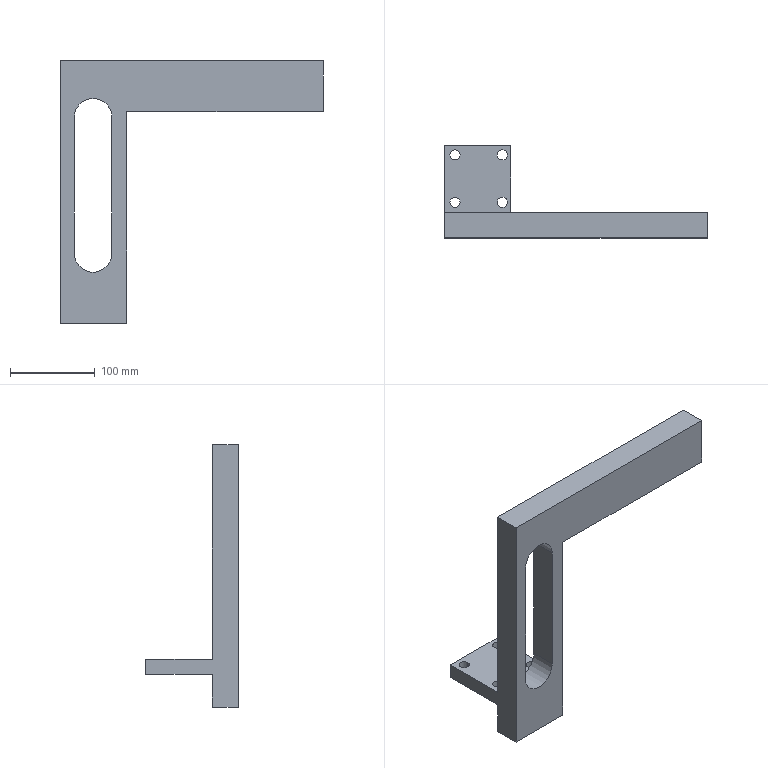Component | SolidWorks | PlateLeft-1 | 1 solid | 24 faces | box 310 x 109.58 x 310 mm | volume 1001004 mm3 | plane 14 | cylinder 10 | commonest cylinder face diameters 12 x8 44.62 x2
build123d program:
from build123d import *

# Parameters (mm, degrees)
SKETCH1_W           = 60
SKETCH1_H           = 30.58
BOSS_EXTRUDE1_DEPTH = 310
SKETCH2_W           = 78
SKETCH2_H           = 30.58
BOSS_EXTRUDE2_DEPTH = 250
CUT_EXTRUDE1_DEPTH  = 120
SKETCH4_W           = 18
SKETCH4_H           = 78
BOSS_EXTRUDE3_DEPTH = 79
SKETCH5_R           = 6
CUT_EXTRUDE2_DEPTH  = 39


with BuildPart() as part:
    # Sketch1 → Boss-Extrude1 (new body)
    with BuildSketch(Plane.XY):
        with Locations((-147.351, -28.878)):
            Rectangle(SKETCH1_W, SKETCH1_H)
    extrude(amount=BOSS_EXTRUDE1_DEPTH)

    # Sketch2 → Boss-Extrude2 (add)
    with BuildSketch(Plane.ZY.offset(177.351)):
        with Locations((271, -28.878)):
            Rectangle(SKETCH2_W, SKETCH2_H)
    extrude(amount=BOSS_EXTRUDE2_DEPTH)

    # Sketch3 → Cut-Extrude1 (cut)
    with BuildSketch(Plane(origin=(0, -13.588, 0), x_dir=(1, 0, 0), z_dir=(0, 1, 0))):
        with BuildLine():
            Line((-344.724, -249.496), (-184.183, -249.496))
            ThreePointArc((-184.183, -249.496), (-161.873, -271.806), (-184.183, -294.116))
            Line((-184.183, -294.116), (-344.724, -294.116))
            ThreePointArc((-344.724, -294.116), (-367.034, -271.806), (-344.724, -249.496))
        make_face()
    extrude(amount=-CUT_EXTRUDE1_DEPTH, mode=Mode.SUBTRACT)

    # Sketch4 → Boss-Extrude3 (add)
    with BuildSketch(Plane(origin=(0, -13.588, 0), x_dir=(1, 0, 0), z_dir=(0, 1, 0))):
        with Locations((-379.672, -271)):
            Rectangle(SKETCH4_W, SKETCH4_H)
    extrude(amount=BOSS_EXTRUDE3_DEPTH)

    # Sketch5 → Cut-Extrude2 (cut)
    with BuildSketch(Plane.ZY.offset(388.672)):
        with Locations((242, 54.412)):
            Circle(SKETCH5_R)
        with Locations((298, 54.412)):
            Circle(SKETCH5_R)
        with Locations((242, -1.588)):
            Circle(SKETCH5_R)
        with Locations((298, -1.588)):
            Circle(SKETCH5_R)
    extrude(amount=-CUT_EXTRUDE2_DEPTH, mode=Mode.SUBTRACT)


solid = part.part

# Placed as in the assembly
solid = solid.moved(Location((89.443, 0, 0), (0, -90, 0)))
STEP:
#1=CARTESIAN_POINT('',(-7.975,2.142,-14.593));
#2=VERTEX_POINT('',#1);
#3=CARTESIAN_POINT('',(-8.447,2.142,-14.593));
#4=VERTEX_POINT('',#3);
#5=CARTESIAN_POINT('',(-8.211,2.142,-14.593));
#6=DIRECTION('',(0.,0.,-1.));
#7=DIRECTION('',(-1.,0.,0.));
#8=AXIS2_PLACEMENT_3D('',#5,#6,#7);
#9=CIRCLE('',#8,0.2362);
#10=EDGE_CURVE('',#2,#4,#9,.T.);
#11=ORIENTED_EDGE('',*,*,#10,.F.);
#12=CARTESIAN_POINT('',(-7.975,2.142,-15.302));
#13=VERTEX_POINT('',#12);
#14=CARTESIAN_POINT('',(-7.975,2.142,-13.767));
#15=DIRECTION('',(0.,0.,-1.));
#16=VECTOR('',#15,39.37);
#17=LINE('',#14,#16);
#18=EDGE_CURVE('',#2,#13,#17,.T.);
#19=ORIENTED_EDGE('',*,*,#18,.T.);
#20=CARTESIAN_POINT('',(-8.447,2.142,-15.302));
#21=VERTEX_POINT('',#20);
#22=CARTESIAN_POINT('',(-8.211,2.142,-15.302));
#23=DIRECTION('',(0.,0.,-1.));
#24=DIRECTION('',(-1.,0.,0.));
#25=AXIS2_PLACEMENT_3D('',#22,#23,#24);
#26=CIRCLE('',#25,0.2362);
#27=EDGE_CURVE('',#13,#21,#26,.T.);
#28=ORIENTED_EDGE('',*,*,#27,.T.);
#29=CARTESIAN_POINT('',(-8.447,2.142,-13.767));
#30=DIRECTION('',(0.,0.,-1.));
#31=VECTOR('',#30,39.37);
#32=LINE('',#29,#31);
#33=EDGE_CURVE('',#4,#21,#32,.T.);
#34=ORIENTED_EDGE('',*,*,#33,.F.);
#35=EDGE_LOOP('',(#11,#19,#28,#34));
#36=FACE_OUTER_BOUND('',#35,.T.);
#37=CARTESIAN_POINT('',(-8.211,2.142,-13.767));
#38=DIRECTION('',(0.,0.,-1.));
#39=DIRECTION('',(-1.,0.,0.));
#40=AXIS2_PLACEMENT_3D('',#37,#38,#39);
#41=CYLINDRICAL_SURFACE('',#40,0.2362);
#42=ADVANCED_FACE('',(#36),#41,.F.);
#43=CARTESIAN_POINT('',(-5.77,-0.06252,-14.593));
#44=VERTEX_POINT('',#43);
#45=CARTESIAN_POINT('',(-6.242,-0.06252,-14.593));
#46=VERTEX_POINT('',#45);
#47=CARTESIAN_POINT('',(-6.006,-0.06252,-14.593));
#48=DIRECTION('',(0.,0.,-1.));
#49=DIRECTION('',(-1.,0.,0.));
#50=AXIS2_PLACEMENT_3D('',#47,#48,#49);
#51=CIRCLE('',#50,0.2362);
#52=EDGE_CURVE('',#44,#46,#51,.T.);
#53=ORIENTED_EDGE('',*,*,#52,.F.);
#54=CARTESIAN_POINT('',(-5.77,-0.06252,-15.302));
#55=VERTEX_POINT('',#54);
#56=CARTESIAN_POINT('',(-5.77,-0.06252,-13.767));
#57=DIRECTION('',(0.,0.,-1.));
#58=VECTOR('',#57,39.37);
#59=LINE('',#56,#58);
#60=EDGE_CURVE('',#44,#55,#59,.T.);
#61=ORIENTED_EDGE('',*,*,#60,.T.);
#62=CARTESIAN_POINT('',(-6.242,-0.06252,-15.302));
#63=VERTEX_POINT('',#62);
#64=CARTESIAN_POINT('',(-6.006,-0.06252,-15.302));
#65=DIRECTION('',(0.,0.,-1.));
#66=DIRECTION('',(-1.,0.,0.));
#67=AXIS2_PLACEMENT_3D('',#64,#65,#66);
#68=CIRCLE('',#67,0.2362);
#69=EDGE_CURVE('',#55,#63,#68,.T.);
#70=ORIENTED_EDGE('',*,*,#69,.T.);
#71=CARTESIAN_POINT('',(-6.242,-0.06252,-13.767));
#72=DIRECTION('',(0.,0.,-1.));
#73=VECTOR('',#72,39.37);
#74=LINE('',#71,#73);
#75=EDGE_CURVE('',#46,#63,#74,.T.);
#76=ORIENTED_EDGE('',*,*,#75,.F.);
#77=EDGE_LOOP('',(#53,#61,#70,#76));
#78=FACE_OUTER_BOUND('',#77,.T.);
#79=CARTESIAN_POINT('',(-6.006,-0.06252,-13.767));
#80=DIRECTION('',(0.,0.,-1.));
#81=DIRECTION('',(-1.,0.,0.));
#82=AXIS2_PLACEMENT_3D('',#79,#80,#81);
#83=CYLINDRICAL_SURFACE('',#82,0.2362);
#84=ADVANCED_FACE('',(#78),#83,.F.);
#85=CARTESIAN_POINT('',(-7.975,-0.06252,-14.593));
#86=VERTEX_POINT('',#85);
#87=CARTESIAN_POINT('',(-8.447,-0.06252,-14.593));
#88=VERTEX_POINT('',#87);
#89=CARTESIAN_POINT('',(-8.211,-0.06252,-14.593));
#90=DIRECTION('',(0.,0.,-1.));
#91=DIRECTION('',(-1.,0.,0.));
#92=AXIS2_PLACEMENT_3D('',#89,#90,#91);
#93=CIRCLE('',#92,0.2362);
#94=EDGE_CURVE('',#86,#88,#93,.T.);
#95=ORIENTED_EDGE('',*,*,#94,.F.);
#96=CARTESIAN_POINT('',(-7.975,-0.06252,-15.302));
#97=VERTEX_POINT('',#96);
#98=CARTESIAN_POINT('',(-7.975,-0.06252,-13.767));
#99=DIRECTION('',(0.,0.,-1.));
#100=VECTOR('',#99,39.37);
#101=LINE('',#98,#100);
#102=EDGE_CURVE('',#86,#97,#101,.T.);
#103=ORIENTED_EDGE('',*,*,#102,.T.);
#104=CARTESIAN_POINT('',(-8.447,-0.06252,-15.302));
#105=VERTEX_POINT('',#104);
#106=CARTESIAN_POINT('',(-8.211,-0.06252,-15.302));
#107=DIRECTION('',(0.,0.,-1.));
#108=DIRECTION('',(-1.,0.,0.));
#109=AXIS2_PLACEMENT_3D('',#106,#107,#108);
#110=CIRCLE('',#109,0.2362);
#111=EDGE_CURVE('',#97,#105,#110,.T.);
#112=ORIENTED_EDGE('',*,*,#111,.T.);
#113=CARTESIAN_POINT('',(-8.447,-0.06252,-13.767));
#114=DIRECTION('',(0.,0.,-1.));
#115=VECTOR('',#114,39.37);
#116=LINE('',#113,#115);
#117=EDGE_CURVE('',#88,#105,#116,.T.);
#118=ORIENTED_EDGE('',*,*,#117,.F.);
#119=EDGE_LOOP('',(#95,#103,#112,#118));
#120=FACE_OUTER_BOUND('',#119,.T.);
#121=CARTESIAN_POINT('',(-8.211,-0.06252,-13.767));
#122=DIRECTION('',(0.,0.,-1.));
#123=DIRECTION('',(-1.,0.,0.));
#124=AXIS2_PLACEMENT_3D('',#121,#122,#123);
#125=CYLINDRICAL_SURFACE('',#124,0.2362);
#126=ADVANCED_FACE('',(#120),#125,.F.);
#127=CARTESIAN_POINT('',(-5.77,2.142,-14.593));
#128=VERTEX_POINT('',#127);
#129=CARTESIAN_POINT('',(-6.242,2.142,-14.593));
#130=VERTEX_POINT('',#129);
#131=CARTESIAN_POINT('',(-6.006,2.142,-14.593));
#132=DIRECTION('',(0.,0.,-1.));
#133=DIRECTION('',(-1.,0.,0.));
#134=AXIS2_PLACEMENT_3D('',#131,#132,#133);
#135=CIRCLE('',#134,0.2362);
#136=EDGE_CURVE('',#128,#130,#135,.T.);
#137=ORIENTED_EDGE('',*,*,#136,.F.);
#138=CARTESIAN_POINT('',(-5.77,2.142,-15.302));
#139=VERTEX_POINT('',#138);
#140=CARTESIAN_POINT('',(-5.77,2.142,-13.767));
#141=DIRECTION('',(0.,0.,-1.));
#142=VECTOR('',#141,39.37);
#143=LINE('',#140,#142);
#144=EDGE_CURVE('',#128,#139,#143,.T.);
#145=ORIENTED_EDGE('',*,*,#144,.T.);
#146=CARTESIAN_POINT('',(-6.242,2.142,-15.302));
#147=VERTEX_POINT('',#146);
#148=CARTESIAN_POINT('',(-6.006,2.142,-15.302));
#149=DIRECTION('',(0.,0.,-1.));
#150=DIRECTION('',(-1.,0.,0.));
#151=AXIS2_PLACEMENT_3D('',#148,#149,#150);
#152=CIRCLE('',#151,0.2362);
#153=EDGE_CURVE('',#139,#147,#152,.T.);
#154=ORIENTED_EDGE('',*,*,#153,.T.);
#155=CARTESIAN_POINT('',(-6.242,2.142,-13.767));
#156=DIRECTION('',(0.,0.,-1.));
#157=VECTOR('',#156,39.37);
#158=LINE('',#155,#157);
#159=EDGE_CURVE('',#130,#147,#158,.T.);
#160=ORIENTED_EDGE('',*,*,#159,.F.);
#161=EDGE_LOOP('',(#137,#145,#154,#160));
#162=FACE_OUTER_BOUND('',#161,.T.);
#163=CARTESIAN_POINT('',(-6.006,2.142,-13.767));
#164=DIRECTION('',(0.,0.,-1.));
#165=DIRECTION('',(-1.,0.,0.));
#166=AXIS2_PLACEMENT_3D('',#163,#164,#165);
#167=CYLINDRICAL_SURFACE('',#166,0.2362);
#168=ADVANCED_FACE('',(#162),#167,.F.);
#169=CARTESIAN_POINT('',(-8.058,-0.535,-13.572));
#170=VERTEX_POINT('',#169);
#171=CARTESIAN_POINT('',(-8.058,-0.535,-7.251));
#172=VERTEX_POINT('',#171);
#173=CARTESIAN_POINT('',(-8.058,-0.535,-13.572));
#174=DIRECTION('',(0.,0.,1.));
#175=VECTOR('',#174,39.37);
#176=LINE('',#173,#175);
#177=EDGE_CURVE('',#170,#172,#176,.T.);
#178=ORIENTED_EDGE('',*,*,#177,.F.);
#179=CARTESIAN_POINT('',(-6.301,-0.535,-13.572));
#180=VERTEX_POINT('',#179);
#181=CARTESIAN_POINT('',(-7.18,-0.535,-13.572));
#182=DIRECTION('',(0.,1.,0.));
#183=DIRECTION('',(-1.,0.,0.));
#184=AXIS2_PLACEMENT_3D('',#181,#182,#183);
#185=CIRCLE('',#184,0.8783);
#186=EDGE_CURVE('',#180,#170,#185,.T.);
#187=ORIENTED_EDGE('',*,*,#186,.F.);
#188=CARTESIAN_POINT('',(-6.301,-0.535,-7.251));
#189=VERTEX_POINT('',#188);
#190=CARTESIAN_POINT('',(-6.301,-0.535,-13.572));
#191=DIRECTION('',(0.,0.,-1.));
#192=VECTOR('',#191,39.37);
#193=LINE('',#190,#192);
#194=EDGE_CURVE('',#189,#180,#193,.T.);
#195=ORIENTED_EDGE('',*,*,#194,.F.);
#196=CARTESIAN_POINT('',(-7.18,-0.535,-7.251));
#197=DIRECTION('',(0.,1.,0.));
#198=DIRECTION('',(-1.,0.,0.));
#199=AXIS2_PLACEMENT_3D('',#196,#197,#198);
#200=CIRCLE('',#199,0.8783);
#201=EDGE_CURVE('',#172,#189,#200,.T.);
#202=ORIENTED_EDGE('',*,*,#201,.F.);
#203=EDGE_LOOP('',(#178,#187,#195,#202));
#204=FACE_BOUND('',#203,.T.);
#205=CARTESIAN_POINT('',(-8.683,-0.535,-14.593));
#206=VERTEX_POINT('',#205);
#207=CARTESIAN_POINT('',(-5.612,-0.535,-14.593));
#208=VERTEX_POINT('',#207);
#209=CARTESIAN_POINT('',(-5.612,-0.535,-14.593));
#210=DIRECTION('',(1.,-0.,0.));
#211=VECTOR('',#210,39.37);
#212=LINE('',#209,#211);
#213=EDGE_CURVE('',#206,#208,#212,.T.);
#214=ORIENTED_EDGE('',*,*,#213,.F.);
#215=CARTESIAN_POINT('',(-8.683,-0.535,-4.62));
#216=VERTEX_POINT('',#215);
#217=CARTESIAN_POINT('',(-8.683,-0.535,-6.982));
#218=DIRECTION('',(0.,0.,-1.));
#219=VECTOR('',#218,39.37);
#220=LINE('',#217,#219);
#221=EDGE_CURVE('',#216,#206,#220,.T.);
#222=ORIENTED_EDGE('',*,*,#221,.F.);
#223=CARTESIAN_POINT('',(3.521,-0.535,-4.62));
#224=VERTEX_POINT('',#223);
#225=CARTESIAN_POINT('',(-8.683,-0.535,-4.62));
#226=DIRECTION('',(1.,-0.,0.));
#227=VECTOR('',#226,39.37);
#228=LINE('',#225,#227);
#229=EDGE_CURVE('',#216,#224,#228,.T.);
#230=ORIENTED_EDGE('',*,*,#229,.T.);
#231=CARTESIAN_POINT('',(3.521,-0.535,-6.982));
#232=VERTEX_POINT('',#231);
#233=CARTESIAN_POINT('',(3.521,-0.535,-6.982));
#234=DIRECTION('',(0.,0.,-1.));
#235=VECTOR('',#234,39.37);
#236=LINE('',#233,#235);
#237=EDGE_CURVE('',#224,#232,#236,.T.);
#238=ORIENTED_EDGE('',*,*,#237,.T.);
#239=CARTESIAN_POINT('',(-5.612,-0.535,-6.982));
#240=VERTEX_POINT('',#239);
#241=CARTESIAN_POINT('',(-8.683,-0.535,-6.982));
#242=DIRECTION('',(1.,-0.,0.));
#243=VECTOR('',#242,39.37);
#244=LINE('',#241,#243);
#245=EDGE_CURVE('',#240,#232,#244,.T.);
#246=ORIENTED_EDGE('',*,*,#245,.F.);
#247=CARTESIAN_POINT('',(-5.612,-0.535,-16.825));
#248=DIRECTION('',(0.,0.,1.));
#249=VECTOR('',#248,39.37);
#250=LINE('',#247,#249);
#251=EDGE_CURVE('',#208,#240,#250,.T.);
#252=ORIENTED_EDGE('',*,*,#251,.F.);
#253=EDGE_LOOP('',(#214,#222,#230,#238,#246,#252));
#254=FACE_OUTER_BOUND('',#253,.T.);
#255=CARTESIAN_POINT('',(-8.683,-0.535,-6.982));
#256=DIRECTION('',(-0.,-1.,0.));
#257=DIRECTION('',(1.,-0.,0.));
#258=AXIS2_PLACEMENT_3D('',#255,#256,#257);
#259=PLANE('',#258);
#260=ADVANCED_FACE('',(#204,#254),#259,.F.);
#261=CARTESIAN_POINT('',(-5.612,-0.535,-15.302));
#262=VERTEX_POINT('',#261);
#263=CARTESIAN_POINT('',(-8.683,-0.535,-15.302));
#264=VERTEX_POINT('',#263);
#265=CARTESIAN_POINT('',(-5.612,-0.535,-15.302));
#266=DIRECTION('',(-1.,0.,0.));
#267=VECTOR('',#266,39.37);
#268=LINE('',#265,#267);
#269=EDGE_CURVE('',#262,#264,#268,.T.);
#270=ORIENTED_EDGE('',*,*,#269,.F.);
#271=CARTESIAN_POINT('',(-5.612,-0.535,-16.825));
#272=VERTEX_POINT('',#271);
#273=CARTESIAN_POINT('',(-5.612,-0.535,-16.825));
#274=DIRECTION('',(0.,0.,1.));
#275=VECTOR('',#274,39.37);
#276=LINE('',#273,#275);
#277=EDGE_CURVE('',#272,#262,#276,.T.);
#278=ORIENTED_EDGE('',*,*,#277,.F.);
#279=CARTESIAN_POINT('',(-8.683,-0.535,-16.825));
#280=VERTEX_POINT('',#279);
#281=CARTESIAN_POINT('',(-5.612,-0.535,-16.825));
#282=DIRECTION('',(1.,-0.,0.));
#283=VECTOR('',#282,39.37);
#284=LINE('',#281,#283);
#285=EDGE_CURVE('',#280,#272,#284,.T.);
#286=ORIENTED_EDGE('',*,*,#285,.F.);
#287=CARTESIAN_POINT('',(-8.683,-0.535,-6.982));
#288=DIRECTION('',(0.,0.,-1.));
#289=VECTOR('',#288,39.37);
#290=LINE('',#287,#289);
#291=EDGE_CURVE('',#264,#280,#290,.T.);
#292=ORIENTED_EDGE('',*,*,#291,.F.);
#293=EDGE_LOOP('',(#270,#278,#286,#292));
#294=FACE_OUTER_BOUND('',#293,.T.);
#295=CARTESIAN_POINT('',(-8.683,-0.535,-6.982));
#296=DIRECTION('',(-0.,-1.,0.));
#297=DIRECTION('',(1.,-0.,0.));
#298=AXIS2_PLACEMENT_3D('',#295,#296,#297);
#299=PLANE('',#298);
#300=ADVANCED_FACE('',(#294),#299,.F.);
#301=CARTESIAN_POINT('',(-5.612,-1.739,-6.982));
#302=VERTEX_POINT('',#301);
#303=CARTESIAN_POINT('',(-5.612,-0.535,-6.982));
#304=DIRECTION('',(-0.,-1.,0.));
#305=VECTOR('',#304,39.37);
#306=LINE('',#303,#305);
#307=EDGE_CURVE('',#240,#302,#306,.T.);
#308=ORIENTED_EDGE('',*,*,#307,.F.);
#309=ORIENTED_EDGE('',*,*,#245,.T.);
#310=CARTESIAN_POINT('',(3.521,-1.739,-6.982));
#311=VERTEX_POINT('',#310);
#312=CARTESIAN_POINT('',(3.521,-0.535,-6.982));
#313=DIRECTION('',(-0.,-1.,0.));
#314=VECTOR('',#313,39.37);
#315=LINE('',#312,#314);
#316=EDGE_CURVE('',#232,#311,#315,.T.);
#317=ORIENTED_EDGE('',*,*,#316,.T.);
#318=CARTESIAN_POINT('',(-8.683,-1.739,-6.982));
#319=DIRECTION('',(1.,-0.,0.));
#320=VECTOR('',#319,39.37);
#321=LINE('',#318,#320);
#322=EDGE_CURVE('',#302,#311,#321,.T.);
#323=ORIENTED_EDGE('',*,*,#322,.F.);
#324=EDGE_LOOP('',(#308,#309,#317,#323));
#325=FACE_OUTER_BOUND('',#324,.T.);
#326=CARTESIAN_POINT('',(-8.683,-0.535,-6.982));
#327=DIRECTION('',(0.,0.,1.));
#328=DIRECTION('',(1.,-0.,0.));
#329=AXIS2_PLACEMENT_3D('',#326,#327,#328);
#330=PLANE('',#329);
#331=ADVANCED_FACE('',(#325),#330,.F.);
#332=CARTESIAN_POINT('',(-6.301,-1.739,-7.251));
#333=VERTEX_POINT('',#332);
#334=CARTESIAN_POINT('',(-6.301,-1.739,-13.572));
#335=VERTEX_POINT('',#334);
#336=CARTESIAN_POINT('',(-6.301,-1.739,-6.982));
#337=DIRECTION('',(0.,0.,-1.));
#338=VECTOR('',#337,39.37);
#339=LINE('',#336,#338);
#340=EDGE_CURVE('',#333,#335,#339,.T.);
#341=ORIENTED_EDGE('',*,*,#340,.T.);
#342=CARTESIAN_POINT('',(-8.058,-1.739,-13.572));
#343=VERTEX_POINT('',#342);
#344=CARTESIAN_POINT('',(-7.18,-1.739,-13.572));
#345=DIRECTION('',(0.,1.,0.));
#346=DIRECTION('',(-1.,0.,0.));
#347=AXIS2_PLACEMENT_3D('',#344,#345,#346);
#348=CIRCLE('',#347,0.8783);
#349=EDGE_CURVE('',#335,#343,#348,.T.);
#350=ORIENTED_EDGE('',*,*,#349,.T.);
#351=CARTESIAN_POINT('',(-8.058,-1.739,-7.251));
#352=VERTEX_POINT('',#351);
#353=CARTESIAN_POINT('',(-8.058,-1.739,-6.982));
#354=DIRECTION('',(0.,0.,1.));
#355=VECTOR('',#354,39.37);
#356=LINE('',#353,#355);
#357=EDGE_CURVE('',#343,#352,#356,.T.);
#358=ORIENTED_EDGE('',*,*,#357,.T.);
#359=CARTESIAN_POINT('',(-7.18,-1.739,-7.251));
#360=DIRECTION('',(0.,1.,0.));
#361=DIRECTION('',(-1.,0.,0.));
#362=AXIS2_PLACEMENT_3D('',#359,#360,#361);
#363=CIRCLE('',#362,0.8783);
#364=EDGE_CURVE('',#352,#333,#363,.T.);
#365=ORIENTED_EDGE('',*,*,#364,.T.);
#366=EDGE_LOOP('',(#341,#350,#358,#365));
#367=FACE_BOUND('',#366,.T.);
#368=CARTESIAN_POINT('',(3.521,-1.739,-4.62));
#369=VERTEX_POINT('',#368);
#370=CARTESIAN_POINT('',(3.521,-1.739,-6.982));
#371=DIRECTION('',(0.,0.,1.));
#372=VECTOR('',#371,39.37);
#373=LINE('',#370,#372);
#374=EDGE_CURVE('',#311,#369,#373,.T.);
#375=ORIENTED_EDGE('',*,*,#374,.T.);
#376=CARTESIAN_POINT('',(-8.683,-1.739,-4.62));
#377=VERTEX_POINT('',#376);
#378=CARTESIAN_POINT('',(-8.683,-1.739,-4.62));
#379=DIRECTION('',(1.,-0.,0.));
#380=VECTOR('',#379,39.37);
#381=LINE('',#378,#380);
#382=EDGE_CURVE('',#377,#369,#381,.T.);
#383=ORIENTED_EDGE('',*,*,#382,.F.);
#384=CARTESIAN_POINT('',(-8.683,-1.739,-16.825));
#385=VERTEX_POINT('',#384);
#386=CARTESIAN_POINT('',(-8.683,-1.739,-6.982));
#387=DIRECTION('',(0.,0.,1.));
#388=VECTOR('',#387,39.37);
#389=LINE('',#386,#388);
#390=EDGE_CURVE('',#385,#377,#389,.T.);
#391=ORIENTED_EDGE('',*,*,#390,.F.);
#392=CARTESIAN_POINT('',(-5.612,-1.739,-16.825));
#393=VERTEX_POINT('',#392);
#394=CARTESIAN_POINT('',(-5.612,-1.739,-16.825));
#395=DIRECTION('',(-1.,0.,0.));
#396=VECTOR('',#395,39.37);
#397=LINE('',#394,#396);
#398=EDGE_CURVE('',#393,#385,#397,.T.);
#399=ORIENTED_EDGE('',*,*,#398,.F.);
#400=CARTESIAN_POINT('',(-5.612,-1.739,-16.825));
#401=DIRECTION('',(0.,0.,1.));
#402=VECTOR('',#401,39.37);
#403=LINE('',#400,#402);
#404=EDGE_CURVE('',#393,#302,#403,.T.);
#405=ORIENTED_EDGE('',*,*,#404,.T.);
#406=ORIENTED_EDGE('',*,*,#322,.T.);
#407=EDGE_LOOP('',(#375,#383,#391,#399,#405,#406));
#408=FACE_OUTER_BOUND('',#407,.T.);
#409=CARTESIAN_POINT('',(-8.683,-1.739,-6.982));
#410=DIRECTION('',(0.,1.,0.));
#411=DIRECTION('',(-1.,0.,0.));
#412=AXIS2_PLACEMENT_3D('',#409,#410,#411);
#413=PLANE('',#412);
#414=ADVANCED_FACE('',(#367,#408),#413,.F.);
#415=CARTESIAN_POINT('',(3.521,-0.535,-4.62));
#416=DIRECTION('',(0.,1.,0.));
#417=VECTOR('',#416,39.37);
#418=LINE('',#415,#417);
#419=EDGE_CURVE('',#369,#224,#418,.T.);
#420=ORIENTED_EDGE('',*,*,#419,.T.);
#421=ORIENTED_EDGE('',*,*,#229,.F.);
#422=CARTESIAN_POINT('',(-8.683,-0.535,-4.62));
#423=DIRECTION('',(0.,1.,0.));
#424=VECTOR('',#423,39.37);
#425=LINE('',#422,#424);
#426=EDGE_CURVE('',#377,#216,#425,.T.);
#427=ORIENTED_EDGE('',*,*,#426,.F.);
#428=ORIENTED_EDGE('',*,*,#382,.T.);
#429=EDGE_LOOP('',(#420,#421,#427,#428));
#430=FACE_OUTER_BOUND('',#429,.T.);
#431=CARTESIAN_POINT('',(-8.683,-0.535,-4.62));
#432=DIRECTION('',(0.,0.,-1.));
#433=DIRECTION('',(-1.,0.,0.));
#434=AXIS2_PLACEMENT_3D('',#431,#432,#433);
#435=PLANE('',#434);
#436=ADVANCED_FACE('',(#430),#435,.F.);
#437=ORIENTED_EDGE('',*,*,#221,.T.);
#438=CARTESIAN_POINT('',(-8.683,2.575,-14.593));
#439=VERTEX_POINT('',#438);
#440=CARTESIAN_POINT('',(-8.683,2.575,-14.593));
#441=DIRECTION('',(-0.,-1.,0.));
#442=VECTOR('',#441,39.37);
#443=LINE('',#440,#442);
#444=EDGE_CURVE('',#439,#206,#443,.T.);
#445=ORIENTED_EDGE('',*,*,#444,.F.);
#446=CARTESIAN_POINT('',(-8.683,2.575,-15.302));
#447=VERTEX_POINT('',#446);
#448=CARTESIAN_POINT('',(-8.683,2.575,-14.593));
#449=DIRECTION('',(0.,0.,1.));
#450=VECTOR('',#449,39.37);
#451=LINE('',#448,#450);
#452=EDGE_CURVE('',#447,#439,#451,.T.);
#453=ORIENTED_EDGE('',*,*,#452,.F.);
#454=CARTESIAN_POINT('',(-8.683,2.575,-15.302));
#455=DIRECTION('',(-0.,-1.,0.));
#456=VECTOR('',#455,39.37);
#457=LINE('',#454,#456);
#458=EDGE_CURVE('',#447,#264,#457,.T.);
#459=ORIENTED_EDGE('',*,*,#458,.T.);
#460=ORIENTED_EDGE('',*,*,#291,.T.);
#461=CARTESIAN_POINT('',(-8.683,-0.535,-16.825));
#462=DIRECTION('',(0.,1.,0.));
#463=VECTOR('',#462,39.37);
#464=LINE('',#461,#463);
#465=EDGE_CURVE('',#385,#280,#464,.T.);
#466=ORIENTED_EDGE('',*,*,#465,.F.);
#467=ORIENTED_EDGE('',*,*,#390,.T.);
#468=ORIENTED_EDGE('',*,*,#426,.T.);
#469=EDGE_LOOP('',(#437,#445,#453,#459,#460,#466,#467,#468));
#470=FACE_OUTER_BOUND('',#469,.T.);
#471=CARTESIAN_POINT('',(-8.683,-0.,-0.));
#472=DIRECTION('',(-1.,0.,0.));
#473=DIRECTION('',(0.,0.,1.));
#474=AXIS2_PLACEMENT_3D('',#471,#472,#473);
#475=PLANE('',#474);
#476=ADVANCED_FACE('',(#470),#475,.T.);
#477=ORIENTED_EDGE('',*,*,#316,.F.);
#478=ORIENTED_EDGE('',*,*,#237,.F.);
#479=ORIENTED_EDGE('',*,*,#419,.F.);
#480=ORIENTED_EDGE('',*,*,#374,.F.);
#481=EDGE_LOOP('',(#477,#478,#479,#480));
#482=FACE_OUTER_BOUND('',#481,.T.);
#483=CARTESIAN_POINT('',(3.521,-0.,-0.));
#484=DIRECTION('',(-1.,0.,0.));
#485=DIRECTION('',(0.,0.,1.));
#486=AXIS2_PLACEMENT_3D('',#483,#484,#485);
#487=PLANE('',#486);
#488=ADVANCED_FACE('',(#482),#487,.F.);
#489=ORIENTED_EDGE('',*,*,#307,.T.);
#490=ORIENTED_EDGE('',*,*,#404,.F.);
#491=CARTESIAN_POINT('',(-5.612,-0.535,-16.825));
#492=DIRECTION('',(-0.,-1.,0.));
#493=VECTOR('',#492,39.37);
#494=LINE('',#491,#493);
#495=EDGE_CURVE('',#272,#393,#494,.T.);
#496=ORIENTED_EDGE('',*,*,#495,.F.);
#497=ORIENTED_EDGE('',*,*,#277,.T.);
#498=CARTESIAN_POINT('',(-5.612,2.575,-15.302));
#499=VERTEX_POINT('',#498);
#500=CARTESIAN_POINT('',(-5.612,2.575,-15.302));
#501=DIRECTION('',(-0.,-1.,0.));
#502=VECTOR('',#501,39.37);
#503=LINE('',#500,#502);
#504=EDGE_CURVE('',#499,#262,#503,.T.);
#505=ORIENTED_EDGE('',*,*,#504,.F.);
#506=CARTESIAN_POINT('',(-5.612,2.575,-14.593));
#507=VERTEX_POINT('',#506);
#508=CARTESIAN_POINT('',(-5.612,2.575,-14.593));
#509=DIRECTION('',(0.,0.,-1.));
#510=VECTOR('',#509,39.37);
#511=LINE('',#508,#510);
#512=EDGE_CURVE('',#507,#499,#511,.T.);
#513=ORIENTED_EDGE('',*,*,#512,.F.);
#514=CARTESIAN_POINT('',(-5.612,2.575,-14.593));
#515=DIRECTION('',(-0.,-1.,0.));
#516=VECTOR('',#515,39.37);
#517=LINE('',#514,#516);
#518=EDGE_CURVE('',#507,#208,#517,.T.);
#519=ORIENTED_EDGE('',*,*,#518,.T.);
#520=ORIENTED_EDGE('',*,*,#251,.T.);
#521=EDGE_LOOP('',(#489,#490,#496,#497,#505,#513,#519,#520));
#522=FACE_OUTER_BOUND('',#521,.T.);
#523=CARTESIAN_POINT('',(-5.612,-0.535,-16.825));
#524=DIRECTION('',(-1.,0.,0.));
#525=DIRECTION('',(0.,0.,1.));
#526=AXIS2_PLACEMENT_3D('',#523,#524,#525);
#527=PLANE('',#526);
#528=ADVANCED_FACE('',(#522),#527,.F.);
#529=ORIENTED_EDGE('',*,*,#495,.T.);
#530=ORIENTED_EDGE('',*,*,#398,.T.);
#531=ORIENTED_EDGE('',*,*,#465,.T.);
#532=ORIENTED_EDGE('',*,*,#285,.T.);
#533=EDGE_LOOP('',(#529,#530,#531,#532));
#534=FACE_OUTER_BOUND('',#533,.T.);
#535=CARTESIAN_POINT('',(3.521,-0.,-16.825));
#536=DIRECTION('',(0.,0.,-1.));
#537=DIRECTION('',(-1.,0.,0.));
#538=AXIS2_PLACEMENT_3D('',#535,#536,#537);
#539=PLANE('',#538);
#540=ADVANCED_FACE('',(#534),#539,.T.);
#541=CARTESIAN_POINT('',(-6.301,-5.259,-13.572));
#542=DIRECTION('',(0.,1.,0.));
#543=VECTOR('',#542,39.37);
#544=LINE('',#541,#543);
#545=EDGE_CURVE('',#335,#180,#544,.T.);
#546=ORIENTED_EDGE('',*,*,#545,.T.);
#547=ORIENTED_EDGE('',*,*,#186,.T.);
#548=CARTESIAN_POINT('',(-8.058,-5.259,-13.572));
#549=DIRECTION('',(0.,1.,0.));
#550=VECTOR('',#549,39.37);
#551=LINE('',#548,#550);
#552=EDGE_CURVE('',#343,#170,#551,.T.);
#553=ORIENTED_EDGE('',*,*,#552,.F.);
#554=ORIENTED_EDGE('',*,*,#349,.F.);
#555=EDGE_LOOP('',(#546,#547,#553,#554));
#556=FACE_OUTER_BOUND('',#555,.T.);
#557=CARTESIAN_POINT('',(-7.18,-5.259,-13.572));
#558=DIRECTION('',(0.,1.,0.));
#559=DIRECTION('',(-1.,0.,0.));
#560=AXIS2_PLACEMENT_3D('',#557,#558,#559);
#561=CYLINDRICAL_SURFACE('',#560,0.8783);
#562=ADVANCED_FACE('',(#556),#561,.F.);
#563=CARTESIAN_POINT('',(-6.301,-5.259,-7.251));
#564=DIRECTION('',(0.,1.,0.));
#565=VECTOR('',#564,39.37);
#566=LINE('',#563,#565);
#567=EDGE_CURVE('',#333,#189,#566,.T.);
#568=ORIENTED_EDGE('',*,*,#567,.T.);
#569=ORIENTED_EDGE('',*,*,#194,.T.);
#570=ORIENTED_EDGE('',*,*,#545,.F.);
#571=ORIENTED_EDGE('',*,*,#340,.F.);
#572=EDGE_LOOP('',(#568,#569,#570,#571));
#573=FACE_OUTER_BOUND('',#572,.T.);
#574=CARTESIAN_POINT('',(-6.301,-5.259,-13.572));
#575=DIRECTION('',(1.,-0.,0.));
#576=DIRECTION('',(0.,0.,-1.));
#577=AXIS2_PLACEMENT_3D('',#574,#575,#576);
#578=PLANE('',#577);
#579=ADVANCED_FACE('',(#573),#578,.F.);
#580=CARTESIAN_POINT('',(-8.058,-5.259,-7.251));
#581=DIRECTION('',(0.,1.,0.));
#582=VECTOR('',#581,39.37);
#583=LINE('',#580,#582);
#584=EDGE_CURVE('',#352,#172,#583,.T.);
#585=ORIENTED_EDGE('',*,*,#584,.T.);
#586=ORIENTED_EDGE('',*,*,#201,.T.);
#587=ORIENTED_EDGE('',*,*,#567,.F.);
#588=ORIENTED_EDGE('',*,*,#364,.F.);
#589=EDGE_LOOP('',(#585,#586,#587,#588));
#590=FACE_OUTER_BOUND('',#589,.T.);
#591=CARTESIAN_POINT('',(-7.18,-5.259,-7.251));
#592=DIRECTION('',(0.,1.,0.));
#593=DIRECTION('',(-1.,0.,0.));
#594=AXIS2_PLACEMENT_3D('',#591,#592,#593);
#595=CYLINDRICAL_SURFACE('',#594,0.8783);
#596=ADVANCED_FACE('',(#590),#595,.F.);
#597=ORIENTED_EDGE('',*,*,#552,.T.);
#598=ORIENTED_EDGE('',*,*,#177,.T.);
#599=ORIENTED_EDGE('',*,*,#584,.F.);
#600=ORIENTED_EDGE('',*,*,#357,.F.);
#601=EDGE_LOOP('',(#597,#598,#599,#600));
#602=FACE_OUTER_BOUND('',#601,.T.);
#603=CARTESIAN_POINT('',(-8.058,-5.259,-13.572));
#604=DIRECTION('',(-1.,0.,0.));
#605=DIRECTION('',(0.,0.,1.));
#606=AXIS2_PLACEMENT_3D('',#603,#604,#605);
#607=PLANE('',#606);
#608=ADVANCED_FACE('',(#602),#607,.F.);
#609=CARTESIAN_POINT('',(-8.211,2.142,-14.593));
#610=DIRECTION('',(0.,0.,-1.));
#611=DIRECTION('',(-1.,0.,0.));
#612=AXIS2_PLACEMENT_3D('',#609,#610,#611);
#613=CIRCLE('',#612,0.2362);
#614=EDGE_CURVE('',#4,#2,#613,.T.);
#615=ORIENTED_EDGE('',*,*,#614,.T.);
#616=ORIENTED_EDGE('',*,*,#10,.T.);
#617=EDGE_LOOP('',(#615,#616));
#618=FACE_BOUND('',#617,.T.);
#619=CARTESIAN_POINT('',(-6.006,-0.06252,-14.593));
#620=DIRECTION('',(0.,0.,-1.));
#621=DIRECTION('',(-1.,0.,0.));
#622=AXIS2_PLACEMENT_3D('',#619,#620,#621);
#623=CIRCLE('',#622,0.2362);
#624=EDGE_CURVE('',#46,#44,#623,.T.);
#625=ORIENTED_EDGE('',*,*,#624,.T.);
#626=ORIENTED_EDGE('',*,*,#52,.T.);
#627=EDGE_LOOP('',(#625,#626));
#628=FACE_BOUND('',#627,.T.);
#629=CARTESIAN_POINT('',(-8.211,-0.06252,-14.593));
#630=DIRECTION('',(0.,0.,-1.));
#631=DIRECTION('',(-1.,0.,0.));
#632=AXIS2_PLACEMENT_3D('',#629,#630,#631);
#633=CIRCLE('',#632,0.2362);
#634=EDGE_CURVE('',#88,#86,#633,.T.);
#635=ORIENTED_EDGE('',*,*,#634,.T.);
#636=ORIENTED_EDGE('',*,*,#94,.T.);
#637=EDGE_LOOP('',(#635,#636));
#638=FACE_BOUND('',#637,.T.);
#639=CARTESIAN_POINT('',(-6.006,2.142,-14.593));
#640=DIRECTION('',(0.,0.,-1.));
#641=DIRECTION('',(-1.,0.,0.));
#642=AXIS2_PLACEMENT_3D('',#639,#640,#641);
#643=CIRCLE('',#642,0.2362);
#644=EDGE_CURVE('',#130,#128,#643,.T.);
#645=ORIENTED_EDGE('',*,*,#644,.T.);
#646=ORIENTED_EDGE('',*,*,#136,.T.);
#647=EDGE_LOOP('',(#645,#646));
#648=FACE_BOUND('',#647,.T.);
#649=ORIENTED_EDGE('',*,*,#213,.T.);
#650=ORIENTED_EDGE('',*,*,#518,.F.);
#651=CARTESIAN_POINT('',(-5.612,2.575,-14.593));
#652=DIRECTION('',(1.,-0.,0.));
#653=VECTOR('',#652,39.37);
#654=LINE('',#651,#653);
#655=EDGE_CURVE('',#439,#507,#654,.T.);
#656=ORIENTED_EDGE('',*,*,#655,.F.);
#657=ORIENTED_EDGE('',*,*,#444,.T.);
#658=EDGE_LOOP('',(#649,#650,#656,#657));
#659=FACE_OUTER_BOUND('',#658,.T.);
#660=CARTESIAN_POINT('',(-5.612,2.575,-14.593));
#661=DIRECTION('',(0.,0.,-1.));
#662=DIRECTION('',(-1.,0.,0.));
#663=AXIS2_PLACEMENT_3D('',#660,#661,#662);
#664=PLANE('',#663);
#665=ADVANCED_FACE('',(#618,#628,#638,#648,#659),#664,.F.);
#666=CARTESIAN_POINT('',(-8.211,2.142,-15.302));
#667=DIRECTION('',(0.,0.,-1.));
#668=DIRECTION('',(-1.,0.,0.));
#669=AXIS2_PLACEMENT_3D('',#666,#667,#668);
#670=CIRCLE('',#669,0.2362);
#671=EDGE_CURVE('',#21,#13,#670,.T.);
#672=ORIENTED_EDGE('',*,*,#671,.F.);
#673=ORIENTED_EDGE('',*,*,#27,.F.);
#674=EDGE_LOOP('',(#672,#673));
#675=FACE_BOUND('',#674,.T.);
#676=CARTESIAN_POINT('',(-6.006,-0.06252,-15.302));
#677=DIRECTION('',(0.,0.,-1.));
#678=DIRECTION('',(-1.,0.,0.));
#679=AXIS2_PLACEMENT_3D('',#676,#677,#678);
#680=CIRCLE('',#679,0.2362);
#681=EDGE_CURVE('',#63,#55,#680,.T.);
#682=ORIENTED_EDGE('',*,*,#681,.F.);
#683=ORIENTED_EDGE('',*,*,#69,.F.);
#684=EDGE_LOOP('',(#682,#683));
#685=FACE_BOUND('',#684,.T.);
#686=CARTESIAN_POINT('',(-8.211,-0.06252,-15.302));
#687=DIRECTION('',(0.,0.,-1.));
#688=DIRECTION('',(-1.,0.,0.));
#689=AXIS2_PLACEMENT_3D('',#686,#687,#688);
#690=CIRCLE('',#689,0.2362);
#691=EDGE_CURVE('',#105,#97,#690,.T.);
#692=ORIENTED_EDGE('',*,*,#691,.F.);
#693=ORIENTED_EDGE('',*,*,#111,.F.);
#694=EDGE_LOOP('',(#692,#693));
#695=FACE_BOUND('',#694,.T.);
#696=CARTESIAN_POINT('',(-6.006,2.142,-15.302));
#697=DIRECTION('',(0.,0.,-1.));
#698=DIRECTION('',(-1.,0.,0.));
#699=AXIS2_PLACEMENT_3D('',#696,#697,#698);
#700=CIRCLE('',#699,0.2362);
#701=EDGE_CURVE('',#147,#139,#700,.T.);
#702=ORIENTED_EDGE('',*,*,#701,.F.);
#703=ORIENTED_EDGE('',*,*,#153,.F.);
#704=EDGE_LOOP('',(#702,#703));
#705=FACE_BOUND('',#704,.T.);
#706=ORIENTED_EDGE('',*,*,#269,.T.);
#707=ORIENTED_EDGE('',*,*,#458,.F.);
#708=CARTESIAN_POINT('',(-5.612,2.575,-15.302));
#709=DIRECTION('',(-1.,0.,0.));
#710=VECTOR('',#709,39.37);
#711=LINE('',#708,#710);
#712=EDGE_CURVE('',#499,#447,#711,.T.);
#713=ORIENTED_EDGE('',*,*,#712,.F.);
#714=ORIENTED_EDGE('',*,*,#504,.T.);
#715=EDGE_LOOP('',(#706,#707,#713,#714));
#716=FACE_OUTER_BOUND('',#715,.T.);
#717=CARTESIAN_POINT('',(-5.612,2.575,-15.302));
#718=DIRECTION('',(0.,-0.,1.));
#719=DIRECTION('',(1.,-0.,-0.));
#720=AXIS2_PLACEMENT_3D('',#717,#718,#719);
#721=PLANE('',#720);
#722=ADVANCED_FACE('',(#675,#685,#695,#705,#716),#721,.F.);
#723=ORIENTED_EDGE('',*,*,#655,.T.);
#724=ORIENTED_EDGE('',*,*,#512,.T.);
#725=ORIENTED_EDGE('',*,*,#712,.T.);
#726=ORIENTED_EDGE('',*,*,#452,.T.);
#727=EDGE_LOOP('',(#723,#724,#725,#726));
#728=FACE_OUTER_BOUND('',#727,.T.);
#729=CARTESIAN_POINT('',(3.521,2.575,-0.));
#730=DIRECTION('',(-0.,-1.,0.));
#731=DIRECTION('',(1.,-0.,0.));
#732=AXIS2_PLACEMENT_3D('',#729,#730,#731);
#733=PLANE('',#732);
#734=ADVANCED_FACE('',(#728),#733,.F.);
#735=ORIENTED_EDGE('',*,*,#144,.F.);
#736=ORIENTED_EDGE('',*,*,#644,.F.);
#737=ORIENTED_EDGE('',*,*,#159,.T.);
#738=ORIENTED_EDGE('',*,*,#701,.T.);
#739=EDGE_LOOP('',(#735,#736,#737,#738));
#740=FACE_OUTER_BOUND('',#739,.T.);
#741=CARTESIAN_POINT('',(-6.006,2.142,-13.767));
#742=DIRECTION('',(0.,0.,-1.));
#743=DIRECTION('',(-1.,0.,0.));
#744=AXIS2_PLACEMENT_3D('',#741,#742,#743);
#745=CYLINDRICAL_SURFACE('',#744,0.2362);
#746=ADVANCED_FACE('',(#740),#745,.F.);
#747=ORIENTED_EDGE('',*,*,#102,.F.);
#748=ORIENTED_EDGE('',*,*,#634,.F.);
#749=ORIENTED_EDGE('',*,*,#117,.T.);
#750=ORIENTED_EDGE('',*,*,#691,.T.);
#751=EDGE_LOOP('',(#747,#748,#749,#750));
#752=FACE_OUTER_BOUND('',#751,.T.);
#753=CARTESIAN_POINT('',(-8.211,-0.06252,-13.767));
#754=DIRECTION('',(0.,0.,-1.));
#755=DIRECTION('',(-1.,0.,0.));
#756=AXIS2_PLACEMENT_3D('',#753,#754,#755);
#757=CYLINDRICAL_SURFACE('',#756,0.2362);
#758=ADVANCED_FACE('',(#752),#757,.F.);
#759=ORIENTED_EDGE('',*,*,#60,.F.);
#760=ORIENTED_EDGE('',*,*,#624,.F.);
#761=ORIENTED_EDGE('',*,*,#75,.T.);
#762=ORIENTED_EDGE('',*,*,#681,.T.);
#763=EDGE_LOOP('',(#759,#760,#761,#762));
#764=FACE_OUTER_BOUND('',#763,.T.);
#765=CARTESIAN_POINT('',(-6.006,-0.06252,-13.767));
#766=DIRECTION('',(0.,0.,-1.));
#767=DIRECTION('',(-1.,0.,0.));
#768=AXIS2_PLACEMENT_3D('',#765,#766,#767);
#769=CYLINDRICAL_SURFACE('',#768,0.2362);
#770=ADVANCED_FACE('',(#764),#769,.F.);
#771=ORIENTED_EDGE('',*,*,#18,.F.);
#772=ORIENTED_EDGE('',*,*,#614,.F.);
#773=ORIENTED_EDGE('',*,*,#33,.T.);
#774=ORIENTED_EDGE('',*,*,#671,.T.);
#775=EDGE_LOOP('',(#771,#772,#773,#774));
#776=FACE_OUTER_BOUND('',#775,.T.);
#777=CARTESIAN_POINT('',(-8.211,2.142,-13.767));
#778=DIRECTION('',(0.,0.,-1.));
#779=DIRECTION('',(-1.,0.,0.));
#780=AXIS2_PLACEMENT_3D('',#777,#778,#779);
#781=CYLINDRICAL_SURFACE('',#780,0.2362);
#782=ADVANCED_FACE('',(#776),#781,.F.);
#783=CLOSED_SHELL('',(#42,#84,#126,#168,#260,#300,#331,#414,#436,#476,#488,#528,#540,#562,#579,#596,#608,#665,#722,#734,#746,#758,#770,#782));
#784=MANIFOLD_SOLID_BREP('',#783);
#785=CARTESIAN_POINT('',(0.,0.,0.));
#786=DIRECTION('',(0.,0.,1.));
#787=DIRECTION('',(1.,0.,0.));
#788=AXIS2_PLACEMENT_3D('',#785,#786,#787);
#789=(LENGTH_UNIT()NAMED_UNIT(*)SI_UNIT($,.METRE.));
#790=LENGTH_MEASURE_WITH_UNIT(LENGTH_MEASURE(0.0254),#789);
#791=DIMENSIONAL_EXPONENTS(1.,0.,0.,0.,0.,0.,0.);
#792=(CONVERSION_BASED_UNIT('',#790)LENGTH_UNIT()NAMED_UNIT(#791));
#793=UNCERTAINTY_MEASURE_WITH_UNIT(LENGTH_MEASURE(0.00001),#792,'','');
#794=(NAMED_UNIT(*)PLANE_ANGLE_UNIT()SI_UNIT($,.RADIAN.));
#795=(NAMED_UNIT(*)SI_UNIT($,.STERADIAN.)SOLID_ANGLE_UNIT());
#796=(GEOMETRIC_REPRESENTATION_CONTEXT(3)GLOBAL_UNCERTAINTY_ASSIGNED_CONTEXT((#793))GLOBAL_UNIT_ASSIGNED_CONTEXT((#792,#794,#795))REPRESENTATION_CONTEXT('',''));
#797=ADVANCED_BREP_SHAPE_REPRESENTATION('',(#784,#788),#796);
#798=COLOUR_RGB('',0.7922,0.8196,0.9333);
#799=FILL_AREA_STYLE_COLOUR('',#798);
#800=FILL_AREA_STYLE('',(#799));
#801=SURFACE_STYLE_FILL_AREA(#800);
#802=SURFACE_SIDE_STYLE('',(#801));
#803=SURFACE_STYLE_USAGE(.BOTH.,#802);
#804=PRESENTATION_STYLE_ASSIGNMENT((#803));
#805=STYLED_ITEM('',(#804),#784);
#806=(LENGTH_UNIT()NAMED_UNIT(*)SI_UNIT($,.METRE.));
#807=LENGTH_MEASURE_WITH_UNIT(LENGTH_MEASURE(0.0254),#806);
#808=DIMENSIONAL_EXPONENTS(1.,0.,0.,0.,0.,0.,0.);
#809=(CONVERSION_BASED_UNIT('',#807)LENGTH_UNIT()NAMED_UNIT(#808));
#810=UNCERTAINTY_MEASURE_WITH_UNIT(LENGTH_MEASURE(0.00001),#809,'','');
#811=(NAMED_UNIT(*)PLANE_ANGLE_UNIT()SI_UNIT($,.RADIAN.));
#812=(NAMED_UNIT(*)SI_UNIT($,.STERADIAN.)SOLID_ANGLE_UNIT());
#813=(GEOMETRIC_REPRESENTATION_CONTEXT(3)GLOBAL_UNCERTAINTY_ASSIGNED_CONTEXT((#810))GLOBAL_UNIT_ASSIGNED_CONTEXT((#809,#811,#812))REPRESENTATION_CONTEXT('',''));
#814=MECHANICAL_DESIGN_GEOMETRIC_PRESENTATION_REPRESENTATION('',(#805),#813);
#815=PRESENTATION_LAYER_ASSIGNMENT('','',(#805));